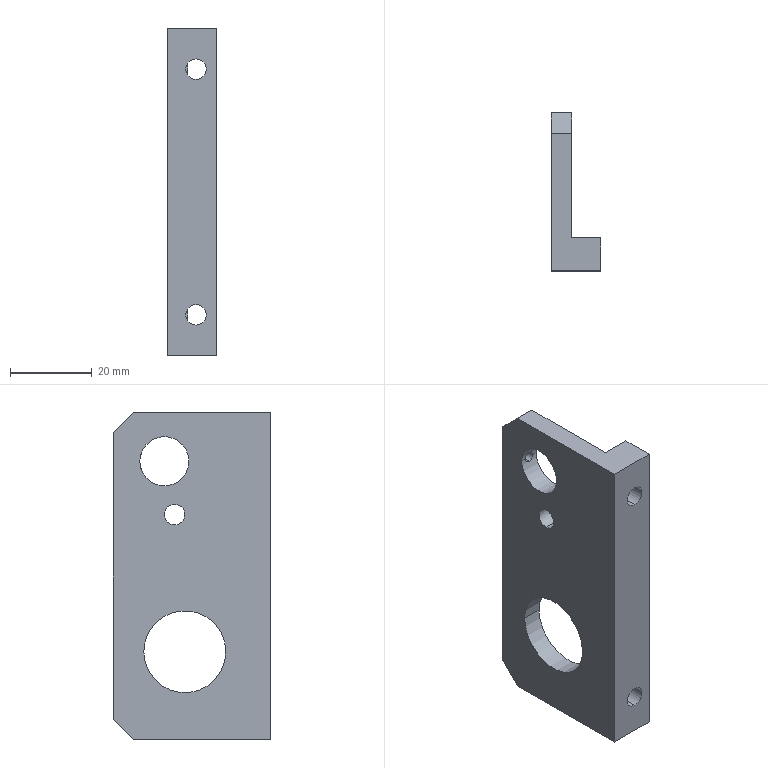Component | SolidWorks | A0116-1 | 1 solid | 24 faces | box 12 x 38.5 x 80 mm | volume 17156 mm3 | cylinder 12 | plane 10 | cone 2 | commonest cylinder face diameters 5 x6 2.5 x2 12 x2 20 x2
build123d program:
from build123d import *

# Parameters (mm, degrees)
BOSS_EXTRUDE1_DEPTH    = 40
SKETCH2_R              = 10
SKETCH2_R_2            = 6
CUT_EXTRUDE1_DEPTH     = 56.958
CHAMFER1_SIZE          = 5
M6_TAPPED_HOLE1_D      = 5
M6_TAPPED_HOLE1_DEPTH  = 17
M6_TAPPED_HOLE1_TIP    = 1.502
M3_TAPPED_HOLE1_REACH  = 58.8
M3_TAPPED_HOLE1_BORE_R = 1.25
M5_TAPPED_HOLE1_D      = 5
M5_TAPPED_HOLE1_DEPTH  = 14
M5_TAPPED_HOLE1_TIP    = 1.502


with BuildPart() as part:
    # Sketch1 → Boss-Extrude1 (new, symmetric)
    with BuildSketch(Plane.XY):
        Polygon((-12, 0), (0, 0), (0, -38.5), (-5, -38.5), (-5, -8), (-12, -8), align=None)
    extrude(amount=BOSS_EXTRUDE1_DEPTH, both=True)

    # Sketch2 → Cut-Extrude1 (cut, through all)
    with BuildSketch(Plane.ZY.offset(5)):
        with Locations(Location((-18.5, -21, 0), (0, 0, 270))):
            Circle(SKETCH2_R)
        with Locations(Location((28, -26, 0), (0, 0, 270))):
            Circle(SKETCH2_R_2)
    extrude(amount=-CUT_EXTRUDE1_DEPTH, mode=Mode.SUBTRACT)

    # Chamfer1
    chamfer1_edges = [part.edges().sort_by_distance(p)[0] for p in [
        (-2.5, -38.5, 40),
        (-2.5, -38.5, -40),
    ]]
    chamfer(chamfer1_edges, length=CHAMFER1_SIZE)

    # M6 Tapped Hole1
    with Locations(Plane(origin=(0, 0, 0), x_dir=(1, 0, 0), z_dir=(0, 1, 0))):
        with Locations((-7, 30), (-7, -30)):
            Hole(M6_TAPPED_HOLE1_D / 2, depth=M6_TAPPED_HOLE1_DEPTH)
            with Locations((0, 0, -(M6_TAPPED_HOLE1_DEPTH + M6_TAPPED_HOLE1_TIP / 2))):  # 118° drill point
                Cone(0, M6_TAPPED_HOLE1_D / 2, M6_TAPPED_HOLE1_TIP, mode=Mode.SUBTRACT)

    # M3 Tapped Hole1 bore → M3 Tapped Hole1 (cut, up to next)
    with BuildSketch(Plane(origin=(0, -38.5, 0), x_dir=(-1, 0, 0), z_dir=(0, -1, 0)), mode=Mode.PRIVATE) as m3_tapped_hole1_sk1:
        with Locations((2.5, -28)):
            Circle(M3_TAPPED_HOLE1_BORE_R)
    m3_tapped_hole1_tool1 = extrude(m3_tapped_hole1_sk1.sketch, amount=-M3_TAPPED_HOLE1_REACH, mode=Mode.PRIVATE) & part.part
    add(m3_tapped_hole1_tool1.solids().sort_by_distance((-2.5, -38.5, 28))[0], mode=Mode.SUBTRACT)

    # M5 Tapped Hole1
    with Locations(Plane(origin=(0, 0, 0), x_dir=(0, 0, -1), z_dir=(1, 0, 0))):
        with Locations((-15, -23.5)):
            Hole(M5_TAPPED_HOLE1_D / 2, depth=M5_TAPPED_HOLE1_DEPTH)
            with Locations((0, 0, -(M5_TAPPED_HOLE1_DEPTH + M5_TAPPED_HOLE1_TIP / 2))):  # 118° drill point
                Cone(0, M5_TAPPED_HOLE1_D / 2, M5_TAPPED_HOLE1_TIP, mode=Mode.SUBTRACT)


solid = part.part

# Placed as in the assembly
solid = solid.moved(Location((-32.619, 0, 60), (0, 0, 180)))
STEP:
#1=COLOUR_RGB('',0.7922,0.8196,0.9333);
#2=FILL_AREA_STYLE_COLOUR('',#1);
#3=FILL_AREA_STYLE('',(#2));
#4=SURFACE_STYLE_FILL_AREA(#3);
#5=SURFACE_SIDE_STYLE('',(#4));
#6=SURFACE_STYLE_USAGE(.BOTH.,#5);
#7=PRESENTATION_STYLE_ASSIGNMENT((#6));
#8=CARTESIAN_POINT('',(-1.087,0.9252,3.051));
#9=VERTEX_POINT('',#8);
#10=CARTESIAN_POINT('',(-1.087,0.9252,2.854));
#11=VERTEX_POINT('',#10);
#12=CARTESIAN_POINT('',(-1.087,0.9252,2.953));
#13=DIRECTION('',(-1.,-0.,0.));
#14=DIRECTION('',(0.,-1.,0.));
#15=AXIS2_PLACEMENT_3D('',#12,#13,#14);
#16=CIRCLE('',#15,0.09843);
#17=EDGE_CURVE('',#9,#11,#16,.T.);
#18=ORIENTED_EDGE('',*,*,#17,.F.);
#19=CARTESIAN_POINT('',(-1.284,0.9252,3.051));
#20=VERTEX_POINT('',#19);
#21=CARTESIAN_POINT('',(-1.284,0.9252,3.051));
#22=DIRECTION('',(-1.,-0.,0.));
#23=VECTOR('',#22,39.37);
#24=LINE('',#21,#23);
#25=EDGE_CURVE('',#9,#20,#24,.T.);
#26=ORIENTED_EDGE('',*,*,#25,.T.);
#27=CARTESIAN_POINT('',(-1.284,0.9252,2.854));
#28=VERTEX_POINT('',#27);
#29=CARTESIAN_POINT('',(-1.284,0.9252,2.953));
#30=DIRECTION('',(-1.,-0.,0.));
#31=DIRECTION('',(-0.,0.,-1.));
#32=AXIS2_PLACEMENT_3D('',#29,#30,#31);
#33=CIRCLE('',#32,0.09843);
#34=EDGE_CURVE('',#20,#28,#33,.T.);
#35=ORIENTED_EDGE('',*,*,#34,.T.);
#36=CARTESIAN_POINT('',(-1.284,0.9252,2.854));
#37=DIRECTION('',(-1.,-0.,0.));
#38=VECTOR('',#37,39.37);
#39=LINE('',#36,#38);
#40=EDGE_CURVE('',#11,#28,#39,.T.);
#41=ORIENTED_EDGE('',*,*,#40,.F.);
#42=EDGE_LOOP('',(#18,#26,#35,#41));
#43=FACE_OUTER_BOUND('',#42,.T.);
#44=CARTESIAN_POINT('',(-1.284,0.9252,2.953));
#45=DIRECTION('',(-1.,-0.,0.));
#46=DIRECTION('',(-0.,0.,-1.));
#47=AXIS2_PLACEMENT_3D('',#44,#45,#46);
#48=CYLINDRICAL_SURFACE('',#47,0.09843);
#49=ADVANCED_FACE('',(#43),#48,.F.);
#50=CARTESIAN_POINT('',(-1.186,1.255,3.514));
#51=VERTEX_POINT('',#50);
#52=CARTESIAN_POINT('',(-1.137,1.26,3.465));
#53=VERTEX_POINT('',#52);
#54=CARTESIAN_POINT('',(-1.186,1.255,3.514));
#55=CARTESIAN_POINT('',(-1.183,1.255,3.514));
#56=CARTESIAN_POINT('',(-1.179,1.255,3.513));
#57=CARTESIAN_POINT('',(-1.173,1.255,3.512));
#58=CARTESIAN_POINT('',(-1.17,1.255,3.511));
#59=CARTESIAN_POINT('',(-1.161,1.256,3.508));
#60=CARTESIAN_POINT('',(-1.156,1.257,3.504));
#61=CARTESIAN_POINT('',(-1.146,1.258,3.495));
#62=CARTESIAN_POINT('',(-1.143,1.259,3.489));
#63=CARTESIAN_POINT('',(-1.138,1.26,3.477));
#64=CARTESIAN_POINT('',(-1.137,1.26,3.471));
#65=CARTESIAN_POINT('',(-1.137,1.26,3.465));
#66=B_SPLINE_CURVE_WITH_KNOTS('',3,(#54,#55,#56,#57,#58,#59,#60,#61,#62,#63,#64,#65),.UNSPECIFIED.,.F.,.F.,(4,2,2,2,2,4),(0.00196,0.002205,0.00245,0.002939,0.003429,0.003919),.UNSPECIFIED.);
#67=EDGE_CURVE('',#51,#53,#66,.T.);
#68=ORIENTED_EDGE('',*,*,#67,.F.);
#69=CARTESIAN_POINT('',(-1.186,1.516,3.514));
#70=VERTEX_POINT('',#69);
#71=CARTESIAN_POINT('',(-1.186,1.516,3.514));
#72=DIRECTION('',(-0.,1.,-0.));
#73=VECTOR('',#72,39.37);
#74=LINE('',#71,#73);
#75=EDGE_CURVE('',#51,#70,#74,.T.);
#76=ORIENTED_EDGE('',*,*,#75,.T.);
#77=CARTESIAN_POINT('',(-1.186,1.516,3.415));
#78=VERTEX_POINT('',#77);
#79=CARTESIAN_POINT('',(-1.186,1.516,3.465));
#80=DIRECTION('',(-0.,1.,-0.));
#81=DIRECTION('',(-0.,0.,-1.));
#82=AXIS2_PLACEMENT_3D('',#79,#80,#81);
#83=CIRCLE('',#82,0.04921);
#84=EDGE_CURVE('',#70,#78,#83,.T.);
#85=ORIENTED_EDGE('',*,*,#84,.T.);
#86=CARTESIAN_POINT('',(-1.186,1.255,3.415));
#87=VERTEX_POINT('',#86);
#88=CARTESIAN_POINT('',(-1.186,1.516,3.415));
#89=DIRECTION('',(-0.,1.,-0.));
#90=VECTOR('',#89,39.37);
#91=LINE('',#88,#90);
#92=EDGE_CURVE('',#87,#78,#91,.T.);
#93=ORIENTED_EDGE('',*,*,#92,.F.);
#94=CARTESIAN_POINT('',(-1.137,1.26,3.465));
#95=CARTESIAN_POINT('',(-1.137,1.26,3.458));
#96=CARTESIAN_POINT('',(-1.138,1.26,3.452));
#97=CARTESIAN_POINT('',(-1.143,1.259,3.44));
#98=CARTESIAN_POINT('',(-1.146,1.258,3.434));
#99=CARTESIAN_POINT('',(-1.156,1.257,3.425));
#100=CARTESIAN_POINT('',(-1.161,1.256,3.422));
#101=CARTESIAN_POINT('',(-1.173,1.255,3.417));
#102=CARTESIAN_POINT('',(-1.179,1.255,3.415));
#103=CARTESIAN_POINT('',(-1.186,1.255,3.415));
#104=B_SPLINE_CURVE_WITH_KNOTS('',3,(#94,#95,#96,#97,#98,#99,#100,#101,#102,#103),.UNSPECIFIED.,.F.,.F.,(4,2,2,2,4),(0.003919,0.004409,0.004899,0.005388,0.005878),.UNSPECIFIED.);
#105=EDGE_CURVE('',#53,#87,#104,.T.);
#106=ORIENTED_EDGE('',*,*,#105,.F.);
#107=EDGE_LOOP('',(#68,#76,#85,#93,#106));
#108=FACE_OUTER_BOUND('',#107,.T.);
#109=CARTESIAN_POINT('',(-1.186,1.516,3.465));
#110=DIRECTION('',(-0.,1.,-0.));
#111=DIRECTION('',(-0.,0.,-1.));
#112=AXIS2_PLACEMENT_3D('',#109,#110,#111);
#113=CYLINDRICAL_SURFACE('',#112,0.04921);
#114=ADVANCED_FACE('',(#108),#113,.F.);
#115=CARTESIAN_POINT('',(-1.009,0.315,1.083));
#116=VERTEX_POINT('',#115);
#117=CARTESIAN_POINT('',(-1.009,0.315,1.28));
#118=VERTEX_POINT('',#117);
#119=CARTESIAN_POINT('',(-1.009,0.315,1.181));
#120=DIRECTION('',(0.,-1.,0.));
#121=DIRECTION('',(1.,0.,-0.));
#122=AXIS2_PLACEMENT_3D('',#119,#120,#121);
#123=CIRCLE('',#122,0.09843);
#124=EDGE_CURVE('',#116,#118,#123,.T.);
#125=ORIENTED_EDGE('',*,*,#124,.F.);
#126=CARTESIAN_POINT('',(-1.009,-0.,1.083));
#127=VERTEX_POINT('',#126);
#128=CARTESIAN_POINT('',(-1.009,-0.,1.083));
#129=DIRECTION('',(0.,-1.,0.));
#130=VECTOR('',#129,39.37);
#131=LINE('',#128,#130);
#132=EDGE_CURVE('',#116,#127,#131,.T.);
#133=ORIENTED_EDGE('',*,*,#132,.T.);
#134=CARTESIAN_POINT('',(-1.009,-0.,1.28));
#135=VERTEX_POINT('',#134);
#136=CARTESIAN_POINT('',(-1.009,-0.,1.181));
#137=DIRECTION('',(0.,-1.,0.));
#138=DIRECTION('',(0.,0.,1.));
#139=AXIS2_PLACEMENT_3D('',#136,#137,#138);
#140=CIRCLE('',#139,0.09843);
#141=EDGE_CURVE('',#127,#135,#140,.T.);
#142=ORIENTED_EDGE('',*,*,#141,.T.);
#143=CARTESIAN_POINT('',(-1.009,-0.,1.28));
#144=DIRECTION('',(0.,-1.,0.));
#145=VECTOR('',#144,39.37);
#146=LINE('',#143,#145);
#147=EDGE_CURVE('',#118,#135,#146,.T.);
#148=ORIENTED_EDGE('',*,*,#147,.F.);
#149=EDGE_LOOP('',(#125,#133,#142,#148));
#150=FACE_OUTER_BOUND('',#149,.T.);
#151=CARTESIAN_POINT('',(-1.009,-0.,1.181));
#152=DIRECTION('',(0.,-1.,0.));
#153=DIRECTION('',(0.,0.,1.));
#154=AXIS2_PLACEMENT_3D('',#151,#152,#153);
#155=CYLINDRICAL_SURFACE('',#154,0.09843);
#156=ADVANCED_FACE('',(#150),#155,.F.);
#157=CARTESIAN_POINT('',(-1.009,0.315,3.445));
#158=VERTEX_POINT('',#157);
#159=CARTESIAN_POINT('',(-1.009,0.315,3.642));
#160=VERTEX_POINT('',#159);
#161=CARTESIAN_POINT('',(-1.009,0.315,3.543));
#162=DIRECTION('',(0.,-1.,0.));
#163=DIRECTION('',(1.,0.,-0.));
#164=AXIS2_PLACEMENT_3D('',#161,#162,#163);
#165=CIRCLE('',#164,0.09843);
#166=EDGE_CURVE('',#158,#160,#165,.T.);
#167=ORIENTED_EDGE('',*,*,#166,.F.);
#168=CARTESIAN_POINT('',(-1.009,-0.,3.445));
#169=VERTEX_POINT('',#168);
#170=CARTESIAN_POINT('',(-1.009,-0.,3.445));
#171=DIRECTION('',(0.,-1.,0.));
#172=VECTOR('',#171,39.37);
#173=LINE('',#170,#172);
#174=EDGE_CURVE('',#158,#169,#173,.T.);
#175=ORIENTED_EDGE('',*,*,#174,.T.);
#176=CARTESIAN_POINT('',(-1.009,-0.,3.642));
#177=VERTEX_POINT('',#176);
#178=CARTESIAN_POINT('',(-1.009,-0.,3.543));
#179=DIRECTION('',(0.,-1.,0.));
#180=DIRECTION('',(0.,0.,1.));
#181=AXIS2_PLACEMENT_3D('',#178,#179,#180);
#182=CIRCLE('',#181,0.09843);
#183=EDGE_CURVE('',#169,#177,#182,.T.);
#184=ORIENTED_EDGE('',*,*,#183,.T.);
#185=CARTESIAN_POINT('',(-1.009,-0.,3.642));
#186=DIRECTION('',(0.,-1.,0.));
#187=VECTOR('',#186,39.37);
#188=LINE('',#185,#187);
#189=EDGE_CURVE('',#160,#177,#188,.T.);
#190=ORIENTED_EDGE('',*,*,#189,.F.);
#191=EDGE_LOOP('',(#167,#175,#184,#190));
#192=FACE_OUTER_BOUND('',#191,.T.);
#193=CARTESIAN_POINT('',(-1.009,-0.,3.543));
#194=DIRECTION('',(0.,-1.,0.));
#195=DIRECTION('',(0.,0.,1.));
#196=AXIS2_PLACEMENT_3D('',#193,#194,#195);
#197=CYLINDRICAL_SURFACE('',#196,0.09843);
#198=ADVANCED_FACE('',(#192),#197,.F.);
#199=CARTESIAN_POINT('',(-1.284,0.7874,3.465));
#200=VERTEX_POINT('',#199);
#201=CARTESIAN_POINT('',(-1.284,1.26,3.465));
#202=VERTEX_POINT('',#201);
#203=CARTESIAN_POINT('',(-1.284,1.024,3.465));
#204=DIRECTION('',(1.,0.,-0.));
#205=DIRECTION('',(-0.,1.,0.));
#206=AXIS2_PLACEMENT_3D('',#203,#204,#205);
#207=CIRCLE('',#206,0.2362);
#208=EDGE_CURVE('',#200,#202,#207,.T.);
#209=ORIENTED_EDGE('',*,*,#208,.F.);
#210=CARTESIAN_POINT('',(-1.087,0.7874,3.465));
#211=VERTEX_POINT('',#210);
#212=CARTESIAN_POINT('',(-1.284,0.7874,3.465));
#213=DIRECTION('',(1.,0.,-0.));
#214=VECTOR('',#213,39.37);
#215=LINE('',#212,#214);
#216=EDGE_CURVE('',#200,#211,#215,.T.);
#217=ORIENTED_EDGE('',*,*,#216,.T.);
#218=CARTESIAN_POINT('',(-1.087,1.26,3.465));
#219=VERTEX_POINT('',#218);
#220=CARTESIAN_POINT('',(-1.087,1.024,3.465));
#221=DIRECTION('',(1.,0.,-0.));
#222=DIRECTION('',(-0.,1.,0.));
#223=AXIS2_PLACEMENT_3D('',#220,#221,#222);
#224=CIRCLE('',#223,0.2362);
#225=EDGE_CURVE('',#211,#219,#224,.T.);
#226=ORIENTED_EDGE('',*,*,#225,.T.);
#227=CARTESIAN_POINT('',(-1.284,1.26,3.465));
#228=DIRECTION('',(1.,0.,-0.));
#229=VECTOR('',#228,39.37);
#230=LINE('',#227,#229);
#231=EDGE_CURVE('',#53,#219,#230,.T.);
#232=ORIENTED_EDGE('',*,*,#231,.F.);
#233=ORIENTED_EDGE('',*,*,#105,.T.);
#234=CARTESIAN_POINT('',(-1.235,1.26,3.465));
#235=VERTEX_POINT('',#234);
#236=CARTESIAN_POINT('',(-1.186,1.255,3.415));
#237=CARTESIAN_POINT('',(-1.192,1.255,3.415));
#238=CARTESIAN_POINT('',(-1.199,1.255,3.417));
#239=CARTESIAN_POINT('',(-1.211,1.256,3.422));
#240=CARTESIAN_POINT('',(-1.216,1.257,3.425));
#241=CARTESIAN_POINT('',(-1.225,1.258,3.434));
#242=CARTESIAN_POINT('',(-1.229,1.259,3.44));
#243=CARTESIAN_POINT('',(-1.234,1.26,3.452));
#244=CARTESIAN_POINT('',(-1.235,1.26,3.458));
#245=CARTESIAN_POINT('',(-1.235,1.26,3.465));
#246=B_SPLINE_CURVE_WITH_KNOTS('',3,(#236,#237,#238,#239,#240,#241,#242,#243,#244,#245),.UNSPECIFIED.,.F.,.F.,(4,2,2,2,4),(0.005878,0.006368,0.006857,0.007347,0.007837),.UNSPECIFIED.);
#247=EDGE_CURVE('',#87,#235,#246,.T.);
#248=ORIENTED_EDGE('',*,*,#247,.T.);
#249=CARTESIAN_POINT('',(-1.284,1.26,3.465));
#250=DIRECTION('',(1.,0.,-0.));
#251=VECTOR('',#250,39.37);
#252=LINE('',#249,#251);
#253=EDGE_CURVE('',#202,#235,#252,.T.);
#254=ORIENTED_EDGE('',*,*,#253,.F.);
#255=EDGE_LOOP('',(#209,#217,#226,#232,#233,#248,#254));
#256=FACE_OUTER_BOUND('',#255,.T.);
#257=CARTESIAN_POINT('',(-1.284,1.024,3.465));
#258=DIRECTION('',(1.,0.,-0.));
#259=DIRECTION('',(-0.,1.,0.));
#260=AXIS2_PLACEMENT_3D('',#257,#258,#259);
#261=CYLINDRICAL_SURFACE('',#260,0.2362);
#262=ADVANCED_FACE('',(#256),#261,.F.);
#263=CARTESIAN_POINT('',(-1.284,0.4331,1.634));
#264=VERTEX_POINT('',#263);
#265=CARTESIAN_POINT('',(-1.284,1.22,1.634));
#266=VERTEX_POINT('',#265);
#267=CARTESIAN_POINT('',(-1.284,0.8268,1.634));
#268=DIRECTION('',(1.,0.,-0.));
#269=DIRECTION('',(-0.,1.,0.));
#270=AXIS2_PLACEMENT_3D('',#267,#268,#269);
#271=CIRCLE('',#270,0.3937);
#272=EDGE_CURVE('',#264,#266,#271,.T.);
#273=ORIENTED_EDGE('',*,*,#272,.F.);
#274=CARTESIAN_POINT('',(-1.087,0.4331,1.634));
#275=VERTEX_POINT('',#274);
#276=CARTESIAN_POINT('',(-1.284,0.4331,1.634));
#277=DIRECTION('',(1.,0.,-0.));
#278=VECTOR('',#277,39.37);
#279=LINE('',#276,#278);
#280=EDGE_CURVE('',#264,#275,#279,.T.);
#281=ORIENTED_EDGE('',*,*,#280,.T.);
#282=CARTESIAN_POINT('',(-1.087,1.22,1.634));
#283=VERTEX_POINT('',#282);
#284=CARTESIAN_POINT('',(-1.087,0.8268,1.634));
#285=DIRECTION('',(1.,0.,-0.));
#286=DIRECTION('',(-0.,1.,0.));
#287=AXIS2_PLACEMENT_3D('',#284,#285,#286);
#288=CIRCLE('',#287,0.3937);
#289=EDGE_CURVE('',#275,#283,#288,.T.);
#290=ORIENTED_EDGE('',*,*,#289,.T.);
#291=CARTESIAN_POINT('',(-1.284,1.22,1.634));
#292=DIRECTION('',(1.,0.,-0.));
#293=VECTOR('',#292,39.37);
#294=LINE('',#291,#293);
#295=EDGE_CURVE('',#266,#283,#294,.T.);
#296=ORIENTED_EDGE('',*,*,#295,.F.);
#297=EDGE_LOOP('',(#273,#281,#290,#296));
#298=FACE_OUTER_BOUND('',#297,.T.);
#299=CARTESIAN_POINT('',(-1.284,0.8268,1.634));
#300=DIRECTION('',(1.,0.,-0.));
#301=DIRECTION('',(-0.,1.,0.));
#302=AXIS2_PLACEMENT_3D('',#299,#300,#301);
#303=CYLINDRICAL_SURFACE('',#302,0.3937);
#304=ADVANCED_FACE('',(#298),#303,.F.);
#305=CARTESIAN_POINT('',(-0.8118,-0.,0.7874));
#306=VERTEX_POINT('',#305);
#307=CARTESIAN_POINT('',(-0.8118,0.315,0.7874));
#308=VERTEX_POINT('',#307);
#309=CARTESIAN_POINT('',(-0.8118,0.315,0.7874));
#310=DIRECTION('',(-0.,1.,-0.));
#311=VECTOR('',#310,39.37);
#312=LINE('',#309,#311);
#313=EDGE_CURVE('',#306,#308,#312,.T.);
#314=ORIENTED_EDGE('',*,*,#313,.T.);
#315=CARTESIAN_POINT('',(-0.8118,0.315,3.937));
#316=VERTEX_POINT('',#315);
#317=CARTESIAN_POINT('',(-0.8118,0.315,3.937));
#318=DIRECTION('',(-0.,-0.,-1.));
#319=VECTOR('',#318,39.37);
#320=LINE('',#317,#319);
#321=EDGE_CURVE('',#316,#308,#320,.T.);
#322=ORIENTED_EDGE('',*,*,#321,.F.);
#323=CARTESIAN_POINT('',(-0.8118,-0.,3.937));
#324=VERTEX_POINT('',#323);
#325=CARTESIAN_POINT('',(-0.8118,0.315,3.937));
#326=DIRECTION('',(-0.,1.,-0.));
#327=VECTOR('',#326,39.37);
#328=LINE('',#325,#327);
#329=EDGE_CURVE('',#324,#316,#328,.T.);
#330=ORIENTED_EDGE('',*,*,#329,.F.);
#331=CARTESIAN_POINT('',(-0.8118,-0.,3.937));
#332=DIRECTION('',(-0.,-0.,-1.));
#333=VECTOR('',#332,39.37);
#334=LINE('',#331,#333);
#335=EDGE_CURVE('',#324,#306,#334,.T.);
#336=ORIENTED_EDGE('',*,*,#335,.T.);
#337=EDGE_LOOP('',(#314,#322,#330,#336));
#338=FACE_OUTER_BOUND('',#337,.T.);
#339=CARTESIAN_POINT('',(-0.8118,0.315,3.937));
#340=DIRECTION('',(-1.,-0.,0.));
#341=DIRECTION('',(-0.,-0.,-1.));
#342=AXIS2_PLACEMENT_3D('',#339,#340,#341);
#343=PLANE('',#342);
#344=ADVANCED_FACE('',(#338),#343,.F.);
#345=CARTESIAN_POINT('',(-1.087,0.315,1.122));
#346=VERTEX_POINT('',#345);
#347=CARTESIAN_POINT('',(-1.087,0.315,0.7874));
#348=VERTEX_POINT('',#347);
#349=CARTESIAN_POINT('',(-1.087,0.315,3.937));
#350=DIRECTION('',(-0.,-0.,-1.));
#351=VECTOR('',#350,39.37);
#352=LINE('',#349,#351);
#353=EDGE_CURVE('',#346,#348,#352,.T.);
#354=ORIENTED_EDGE('',*,*,#353,.F.);
#355=CARTESIAN_POINT('',(-1.009,0.315,1.181));
#356=DIRECTION('',(0.,-1.,0.));
#357=DIRECTION('',(1.,0.,-0.));
#358=AXIS2_PLACEMENT_3D('',#355,#356,#357);
#359=CIRCLE('',#358,0.09843);
#360=EDGE_CURVE('',#346,#116,#359,.T.);
#361=ORIENTED_EDGE('',*,*,#360,.T.);
#362=ORIENTED_EDGE('',*,*,#124,.T.);
#363=CARTESIAN_POINT('',(-1.087,0.315,1.24));
#364=VERTEX_POINT('',#363);
#365=CARTESIAN_POINT('',(-1.009,0.315,1.181));
#366=DIRECTION('',(0.,-1.,0.));
#367=DIRECTION('',(1.,0.,-0.));
#368=AXIS2_PLACEMENT_3D('',#365,#366,#367);
#369=CIRCLE('',#368,0.09843);
#370=EDGE_CURVE('',#118,#364,#369,.T.);
#371=ORIENTED_EDGE('',*,*,#370,.T.);
#372=CARTESIAN_POINT('',(-1.087,0.315,3.484));
#373=VERTEX_POINT('',#372);
#374=CARTESIAN_POINT('',(-1.087,0.315,3.937));
#375=DIRECTION('',(-0.,-0.,-1.));
#376=VECTOR('',#375,39.37);
#377=LINE('',#374,#376);
#378=EDGE_CURVE('',#373,#364,#377,.T.);
#379=ORIENTED_EDGE('',*,*,#378,.F.);
#380=CARTESIAN_POINT('',(-1.009,0.315,3.543));
#381=DIRECTION('',(0.,-1.,0.));
#382=DIRECTION('',(1.,0.,-0.));
#383=AXIS2_PLACEMENT_3D('',#380,#381,#382);
#384=CIRCLE('',#383,0.09843);
#385=EDGE_CURVE('',#373,#158,#384,.T.);
#386=ORIENTED_EDGE('',*,*,#385,.T.);
#387=ORIENTED_EDGE('',*,*,#166,.T.);
#388=CARTESIAN_POINT('',(-1.087,0.315,3.602));
#389=VERTEX_POINT('',#388);
#390=CARTESIAN_POINT('',(-1.009,0.315,3.543));
#391=DIRECTION('',(0.,-1.,0.));
#392=DIRECTION('',(1.,0.,-0.));
#393=AXIS2_PLACEMENT_3D('',#390,#391,#392);
#394=CIRCLE('',#393,0.09843);
#395=EDGE_CURVE('',#160,#389,#394,.T.);
#396=ORIENTED_EDGE('',*,*,#395,.T.);
#397=CARTESIAN_POINT('',(-1.087,0.315,3.937));
#398=VERTEX_POINT('',#397);
#399=CARTESIAN_POINT('',(-1.087,0.315,3.937));
#400=DIRECTION('',(-0.,-0.,-1.));
#401=VECTOR('',#400,39.37);
#402=LINE('',#399,#401);
#403=EDGE_CURVE('',#398,#389,#402,.T.);
#404=ORIENTED_EDGE('',*,*,#403,.F.);
#405=CARTESIAN_POINT('',(-1.087,0.315,3.937));
#406=DIRECTION('',(-1.,-0.,0.));
#407=VECTOR('',#406,39.37);
#408=LINE('',#405,#407);
#409=EDGE_CURVE('',#316,#398,#408,.T.);
#410=ORIENTED_EDGE('',*,*,#409,.F.);
#411=ORIENTED_EDGE('',*,*,#321,.T.);
#412=CARTESIAN_POINT('',(-1.087,0.315,0.7874));
#413=DIRECTION('',(-1.,-0.,0.));
#414=VECTOR('',#413,39.37);
#415=LINE('',#412,#414);
#416=EDGE_CURVE('',#308,#348,#415,.T.);
#417=ORIENTED_EDGE('',*,*,#416,.T.);
#418=EDGE_LOOP('',(#354,#361,#362,#371,#379,#386,#387,#396,#404,#410,#411,#417));
#419=FACE_OUTER_BOUND('',#418,.T.);
#420=CARTESIAN_POINT('',(-1.087,0.315,3.937));
#421=DIRECTION('',(0.,-1.,0.));
#422=DIRECTION('',(1.,0.,-0.));
#423=AXIS2_PLACEMENT_3D('',#420,#421,#422);
#424=PLANE('',#423);
#425=ADVANCED_FACE('',(#419),#424,.F.);
#426=CARTESIAN_POINT('',(-1.087,0.9252,2.953));
#427=DIRECTION('',(-1.,-0.,0.));
#428=DIRECTION('',(0.,-1.,0.));
#429=AXIS2_PLACEMENT_3D('',#426,#427,#428);
#430=CIRCLE('',#429,0.09843);
#431=EDGE_CURVE('',#11,#9,#430,.T.);
#432=ORIENTED_EDGE('',*,*,#431,.T.);
#433=ORIENTED_EDGE('',*,*,#17,.T.);
#434=EDGE_LOOP('',(#432,#433));
#435=FACE_BOUND('',#434,.T.);
#436=CARTESIAN_POINT('',(-1.087,1.024,3.465));
#437=DIRECTION('',(1.,0.,-0.));
#438=DIRECTION('',(-0.,1.,0.));
#439=AXIS2_PLACEMENT_3D('',#436,#437,#438);
#440=CIRCLE('',#439,0.2362);
#441=EDGE_CURVE('',#219,#211,#440,.T.);
#442=ORIENTED_EDGE('',*,*,#441,.F.);
#443=ORIENTED_EDGE('',*,*,#225,.F.);
#444=EDGE_LOOP('',(#442,#443));
#445=FACE_BOUND('',#444,.T.);
#446=CARTESIAN_POINT('',(-1.087,0.8268,1.634));
#447=DIRECTION('',(1.,0.,-0.));
#448=DIRECTION('',(-0.,1.,0.));
#449=AXIS2_PLACEMENT_3D('',#446,#447,#448);
#450=CIRCLE('',#449,0.3937);
#451=EDGE_CURVE('',#283,#275,#450,.T.);
#452=ORIENTED_EDGE('',*,*,#451,.F.);
#453=ORIENTED_EDGE('',*,*,#289,.F.);
#454=EDGE_LOOP('',(#452,#453));
#455=FACE_BOUND('',#454,.T.);
#456=CARTESIAN_POINT('',(-1.087,0.6693,1.24));
#457=VERTEX_POINT('',#456);
#458=CARTESIAN_POINT('',(-1.087,0.6693,1.122));
#459=VERTEX_POINT('',#458);
#460=CARTESIAN_POINT('',(-1.087,0.6693,1.24));
#461=CARTESIAN_POINT('',(-1.087,0.6727,1.231));
#462=CARTESIAN_POINT('',(-1.087,0.6757,1.221));
#463=CARTESIAN_POINT('',(-1.087,0.6799,1.201));
#464=CARTESIAN_POINT('',(-1.087,0.6811,1.191));
#465=CARTESIAN_POINT('',(-1.087,0.6811,1.176));
#466=CARTESIAN_POINT('',(-1.087,0.6808,1.171));
#467=CARTESIAN_POINT('',(-1.087,0.6797,1.161));
#468=CARTESIAN_POINT('',(-1.087,0.6789,1.156));
#469=CARTESIAN_POINT('',(-1.087,0.6757,1.141));
#470=CARTESIAN_POINT('',(-1.087,0.6727,1.132));
#471=CARTESIAN_POINT('',(-1.087,0.6693,1.122));
#472=B_SPLINE_CURVE_WITH_KNOTS('',3,(#460,#461,#462,#463,#464,#465,#466,#467,#468,#469,#470,#471),.UNSPECIFIED.,.F.,.F.,(4,2,2,2,2,4),(0.00544,0.006204,0.006968,0.00735,0.007733,0.008497),.UNSPECIFIED.);
#473=EDGE_CURVE('',#457,#459,#472,.T.);
#474=ORIENTED_EDGE('',*,*,#473,.T.);
#475=CARTESIAN_POINT('',(-1.087,-0.,1.122));
#476=DIRECTION('',(0.,-1.,0.));
#477=VECTOR('',#476,39.37);
#478=LINE('',#475,#477);
#479=EDGE_CURVE('',#459,#346,#478,.T.);
#480=ORIENTED_EDGE('',*,*,#479,.T.);
#481=ORIENTED_EDGE('',*,*,#353,.T.);
#482=CARTESIAN_POINT('',(-1.087,1.319,0.7874));
#483=VERTEX_POINT('',#482);
#484=CARTESIAN_POINT('',(-1.087,1.516,0.7874));
#485=DIRECTION('',(-0.,1.,-0.));
#486=VECTOR('',#485,39.37);
#487=LINE('',#484,#486);
#488=EDGE_CURVE('',#348,#483,#487,.T.);
#489=ORIENTED_EDGE('',*,*,#488,.T.);
#490=CARTESIAN_POINT('',(-1.087,1.516,0.9843));
#491=VERTEX_POINT('',#490);
#492=CARTESIAN_POINT('',(-1.087,1.516,0.9843));
#493=DIRECTION('',(0.,0.7071,0.7071));
#494=VECTOR('',#493,39.37);
#495=LINE('',#492,#494);
#496=EDGE_CURVE('',#483,#491,#495,.T.);
#497=ORIENTED_EDGE('',*,*,#496,.T.);
#498=CARTESIAN_POINT('',(-1.087,1.516,3.74));
#499=VERTEX_POINT('',#498);
#500=CARTESIAN_POINT('',(-1.087,1.516,3.937));
#501=DIRECTION('',(-0.,-0.,-1.));
#502=VECTOR('',#501,39.37);
#503=LINE('',#500,#502);
#504=EDGE_CURVE('',#499,#491,#503,.T.);
#505=ORIENTED_EDGE('',*,*,#504,.F.);
#506=CARTESIAN_POINT('',(-1.087,1.319,3.937));
#507=VERTEX_POINT('',#506);
#508=CARTESIAN_POINT('',(-1.087,1.319,3.937));
#509=DIRECTION('',(0.,-0.7071,0.7071));
#510=VECTOR('',#509,39.37);
#511=LINE('',#508,#510);
#512=EDGE_CURVE('',#499,#507,#511,.T.);
#513=ORIENTED_EDGE('',*,*,#512,.T.);
#514=CARTESIAN_POINT('',(-1.087,1.516,3.937));
#515=DIRECTION('',(-0.,1.,-0.));
#516=VECTOR('',#515,39.37);
#517=LINE('',#514,#516);
#518=EDGE_CURVE('',#398,#507,#517,.T.);
#519=ORIENTED_EDGE('',*,*,#518,.F.);
#520=ORIENTED_EDGE('',*,*,#403,.T.);
#521=CARTESIAN_POINT('',(-1.087,0.6693,3.602));
#522=VERTEX_POINT('',#521);
#523=CARTESIAN_POINT('',(-1.087,-0.,3.602));
#524=DIRECTION('',(-0.,1.,-0.));
#525=VECTOR('',#524,39.37);
#526=LINE('',#523,#525);
#527=EDGE_CURVE('',#389,#522,#526,.T.);
#528=ORIENTED_EDGE('',*,*,#527,.T.);
#529=CARTESIAN_POINT('',(-1.087,0.6693,3.484));
#530=VERTEX_POINT('',#529);
#531=CARTESIAN_POINT('',(-1.087,0.6693,3.602));
#532=CARTESIAN_POINT('',(-1.087,0.6727,3.593));
#533=CARTESIAN_POINT('',(-1.087,0.6757,3.583));
#534=CARTESIAN_POINT('',(-1.087,0.6799,3.564));
#535=CARTESIAN_POINT('',(-1.087,0.6811,3.554));
#536=CARTESIAN_POINT('',(-1.087,0.6811,3.538));
#537=CARTESIAN_POINT('',(-1.087,0.6808,3.533));
#538=CARTESIAN_POINT('',(-1.087,0.6797,3.523));
#539=CARTESIAN_POINT('',(-1.087,0.6789,3.518));
#540=CARTESIAN_POINT('',(-1.087,0.6757,3.503));
#541=CARTESIAN_POINT('',(-1.087,0.6727,3.494));
#542=CARTESIAN_POINT('',(-1.087,0.6693,3.484));
#543=B_SPLINE_CURVE_WITH_KNOTS('',3,(#531,#532,#533,#534,#535,#536,#537,#538,#539,#540,#541,#542),.UNSPECIFIED.,.F.,.F.,(4,2,2,2,2,4),(0.00544,0.006204,0.006968,0.00735,0.007733,0.008497),.UNSPECIFIED.);
#544=EDGE_CURVE('',#522,#530,#543,.T.);
#545=ORIENTED_EDGE('',*,*,#544,.T.);
#546=CARTESIAN_POINT('',(-1.087,-0.,3.484));
#547=DIRECTION('',(0.,-1.,0.));
#548=VECTOR('',#547,39.37);
#549=LINE('',#546,#548);
#550=EDGE_CURVE('',#530,#373,#549,.T.);
#551=ORIENTED_EDGE('',*,*,#550,.T.);
#552=ORIENTED_EDGE('',*,*,#378,.T.);
#553=CARTESIAN_POINT('',(-1.087,-0.,1.24));
#554=DIRECTION('',(-0.,1.,-0.));
#555=VECTOR('',#554,39.37);
#556=LINE('',#553,#555);
#557=EDGE_CURVE('',#364,#457,#556,.T.);
#558=ORIENTED_EDGE('',*,*,#557,.T.);
#559=EDGE_LOOP('',(#474,#480,#481,#489,#497,#505,#513,#519,#520,#528,#545,#551,#552,#558));
#560=FACE_OUTER_BOUND('',#559,.T.);
#561=CARTESIAN_POINT('',(-1.087,1.516,3.937));
#562=DIRECTION('',(-1.,-0.,0.));
#563=DIRECTION('',(0.,-1.,0.));
#564=AXIS2_PLACEMENT_3D('',#561,#562,#563);
#565=PLANE('',#564);
#566=ADVANCED_FACE('',(#435,#445,#455,#560),#565,.F.);
#567=CARTESIAN_POINT('',(-1.186,1.516,3.465));
#568=DIRECTION('',(-0.,1.,-0.));
#569=DIRECTION('',(-0.,0.,-1.));
#570=AXIS2_PLACEMENT_3D('',#567,#568,#569);
#571=CIRCLE('',#570,0.04921);
#572=EDGE_CURVE('',#78,#70,#571,.T.);
#573=ORIENTED_EDGE('',*,*,#572,.F.);
#574=ORIENTED_EDGE('',*,*,#84,.F.);
#575=EDGE_LOOP('',(#573,#574));
#576=FACE_BOUND('',#575,.T.);
#577=CARTESIAN_POINT('',(-1.284,1.516,3.74));
#578=VERTEX_POINT('',#577);
#579=CARTESIAN_POINT('',(-1.284,1.516,0.9843));
#580=VERTEX_POINT('',#579);
#581=CARTESIAN_POINT('',(-1.284,1.516,3.937));
#582=DIRECTION('',(-0.,-0.,-1.));
#583=VECTOR('',#582,39.37);
#584=LINE('',#581,#583);
#585=EDGE_CURVE('',#578,#580,#584,.T.);
#586=ORIENTED_EDGE('',*,*,#585,.F.);
#587=CARTESIAN_POINT('',(-1.284,1.516,3.74));
#588=DIRECTION('',(1.,-0.,-0.));
#589=VECTOR('',#588,39.37);
#590=LINE('',#587,#589);
#591=EDGE_CURVE('',#578,#499,#590,.T.);
#592=ORIENTED_EDGE('',*,*,#591,.T.);
#593=ORIENTED_EDGE('',*,*,#504,.T.);
#594=CARTESIAN_POINT('',(-1.284,1.516,0.9843));
#595=DIRECTION('',(-1.,0.,0.));
#596=VECTOR('',#595,39.37);
#597=LINE('',#594,#596);
#598=EDGE_CURVE('',#491,#580,#597,.T.);
#599=ORIENTED_EDGE('',*,*,#598,.T.);
#600=EDGE_LOOP('',(#586,#592,#593,#599));
#601=FACE_OUTER_BOUND('',#600,.T.);
#602=CARTESIAN_POINT('',(-1.284,1.516,3.937));
#603=DIRECTION('',(-0.,-1.,0.));
#604=DIRECTION('',(1.,-0.,-0.));
#605=AXIS2_PLACEMENT_3D('',#602,#603,#604);
#606=PLANE('',#605);
#607=ADVANCED_FACE('',(#576,#601),#606,.F.);
#608=CARTESIAN_POINT('',(-1.284,0.9252,2.953));
#609=DIRECTION('',(-1.,-0.,0.));
#610=DIRECTION('',(-0.,0.,-1.));
#611=AXIS2_PLACEMENT_3D('',#608,#609,#610);
#612=CIRCLE('',#611,0.09843);
#613=EDGE_CURVE('',#28,#20,#612,.T.);
#614=ORIENTED_EDGE('',*,*,#613,.F.);
#615=ORIENTED_EDGE('',*,*,#34,.F.);
#616=EDGE_LOOP('',(#614,#615));
#617=FACE_BOUND('',#616,.T.);
#618=CARTESIAN_POINT('',(-1.284,1.024,3.465));
#619=DIRECTION('',(1.,0.,-0.));
#620=DIRECTION('',(-0.,1.,0.));
#621=AXIS2_PLACEMENT_3D('',#618,#619,#620);
#622=CIRCLE('',#621,0.2362);
#623=EDGE_CURVE('',#202,#200,#622,.T.);
#624=ORIENTED_EDGE('',*,*,#623,.T.);
#625=ORIENTED_EDGE('',*,*,#208,.T.);
#626=EDGE_LOOP('',(#624,#625));
#627=FACE_BOUND('',#626,.T.);
#628=CARTESIAN_POINT('',(-1.284,0.8268,1.634));
#629=DIRECTION('',(1.,0.,-0.));
#630=DIRECTION('',(-0.,1.,0.));
#631=AXIS2_PLACEMENT_3D('',#628,#629,#630);
#632=CIRCLE('',#631,0.3937);
#633=EDGE_CURVE('',#266,#264,#632,.T.);
#634=ORIENTED_EDGE('',*,*,#633,.T.);
#635=ORIENTED_EDGE('',*,*,#272,.T.);
#636=EDGE_LOOP('',(#634,#635));
#637=FACE_BOUND('',#636,.T.);
#638=CARTESIAN_POINT('',(-1.284,1.319,3.937));
#639=VERTEX_POINT('',#638);
#640=CARTESIAN_POINT('',(-1.284,-0.,3.937));
#641=VERTEX_POINT('',#640);
#642=CARTESIAN_POINT('',(-1.284,-0.,3.937));
#643=DIRECTION('',(0.,-1.,0.));
#644=VECTOR('',#643,39.37);
#645=LINE('',#642,#644);
#646=EDGE_CURVE('',#639,#641,#645,.T.);
#647=ORIENTED_EDGE('',*,*,#646,.F.);
#648=CARTESIAN_POINT('',(-1.284,1.319,3.937));
#649=DIRECTION('',(-0.,0.7071,-0.7071));
#650=VECTOR('',#649,39.37);
#651=LINE('',#648,#650);
#652=EDGE_CURVE('',#639,#578,#651,.T.);
#653=ORIENTED_EDGE('',*,*,#652,.T.);
#654=ORIENTED_EDGE('',*,*,#585,.T.);
#655=CARTESIAN_POINT('',(-1.284,1.319,0.7874));
#656=VERTEX_POINT('',#655);
#657=CARTESIAN_POINT('',(-1.284,1.516,0.9843));
#658=DIRECTION('',(-0.,-0.7071,-0.7071));
#659=VECTOR('',#658,39.37);
#660=LINE('',#657,#659);
#661=EDGE_CURVE('',#580,#656,#660,.T.);
#662=ORIENTED_EDGE('',*,*,#661,.T.);
#663=CARTESIAN_POINT('',(-1.284,-0.,0.7874));
#664=VERTEX_POINT('',#663);
#665=CARTESIAN_POINT('',(-1.284,-0.,0.7874));
#666=DIRECTION('',(0.,-1.,0.));
#667=VECTOR('',#666,39.37);
#668=LINE('',#665,#667);
#669=EDGE_CURVE('',#656,#664,#668,.T.);
#670=ORIENTED_EDGE('',*,*,#669,.T.);
#671=CARTESIAN_POINT('',(-1.284,-0.,3.937));
#672=DIRECTION('',(-0.,-0.,-1.));
#673=VECTOR('',#672,39.37);
#674=LINE('',#671,#673);
#675=EDGE_CURVE('',#641,#664,#674,.T.);
#676=ORIENTED_EDGE('',*,*,#675,.F.);
#677=EDGE_LOOP('',(#647,#653,#654,#662,#670,#676));
#678=FACE_OUTER_BOUND('',#677,.T.);
#679=CARTESIAN_POINT('',(-1.284,-0.,3.937));
#680=DIRECTION('',(1.,0.,-0.));
#681=DIRECTION('',(-0.,1.,-0.));
#682=AXIS2_PLACEMENT_3D('',#679,#680,#681);
#683=PLANE('',#682);
#684=ADVANCED_FACE('',(#617,#627,#637,#678),#683,.F.);
#685=CARTESIAN_POINT('',(-1.009,-0.,1.181));
#686=DIRECTION('',(0.,-1.,0.));
#687=DIRECTION('',(0.,0.,1.));
#688=AXIS2_PLACEMENT_3D('',#685,#686,#687);
#689=CIRCLE('',#688,0.09843);
#690=EDGE_CURVE('',#135,#127,#689,.T.);
#691=ORIENTED_EDGE('',*,*,#690,.F.);
#692=ORIENTED_EDGE('',*,*,#141,.F.);
#693=EDGE_LOOP('',(#691,#692));
#694=FACE_BOUND('',#693,.T.);
#695=CARTESIAN_POINT('',(-1.009,-0.,3.543));
#696=DIRECTION('',(0.,-1.,0.));
#697=DIRECTION('',(0.,0.,1.));
#698=AXIS2_PLACEMENT_3D('',#695,#696,#697);
#699=CIRCLE('',#698,0.09843);
#700=EDGE_CURVE('',#177,#169,#699,.T.);
#701=ORIENTED_EDGE('',*,*,#700,.F.);
#702=ORIENTED_EDGE('',*,*,#183,.F.);
#703=EDGE_LOOP('',(#701,#702));
#704=FACE_BOUND('',#703,.T.);
#705=CARTESIAN_POINT('',(-0.8118,-0.,0.7874));
#706=DIRECTION('',(1.,0.,-0.));
#707=VECTOR('',#706,39.37);
#708=LINE('',#705,#707);
#709=EDGE_CURVE('',#664,#306,#708,.T.);
#710=ORIENTED_EDGE('',*,*,#709,.T.);
#711=ORIENTED_EDGE('',*,*,#335,.F.);
#712=CARTESIAN_POINT('',(-0.8118,-0.,3.937));
#713=DIRECTION('',(1.,0.,-0.));
#714=VECTOR('',#713,39.37);
#715=LINE('',#712,#714);
#716=EDGE_CURVE('',#641,#324,#715,.T.);
#717=ORIENTED_EDGE('',*,*,#716,.F.);
#718=ORIENTED_EDGE('',*,*,#675,.T.);
#719=EDGE_LOOP('',(#710,#711,#717,#718));
#720=FACE_OUTER_BOUND('',#719,.T.);
#721=CARTESIAN_POINT('',(-0.8118,-0.,3.937));
#722=DIRECTION('',(-0.,1.,-0.));
#723=DIRECTION('',(-0.,-0.,-1.));
#724=AXIS2_PLACEMENT_3D('',#721,#722,#723);
#725=PLANE('',#724);
#726=ADVANCED_FACE('',(#694,#704,#720),#725,.F.);
#727=ORIENTED_EDGE('',*,*,#518,.T.);
#728=CARTESIAN_POINT('',(-1.284,1.319,3.937));
#729=DIRECTION('',(-1.,0.,0.));
#730=VECTOR('',#729,39.37);
#731=LINE('',#728,#730);
#732=EDGE_CURVE('',#507,#639,#731,.T.);
#733=ORIENTED_EDGE('',*,*,#732,.T.);
#734=ORIENTED_EDGE('',*,*,#646,.T.);
#735=ORIENTED_EDGE('',*,*,#716,.T.);
#736=ORIENTED_EDGE('',*,*,#329,.T.);
#737=ORIENTED_EDGE('',*,*,#409,.T.);
#738=EDGE_LOOP('',(#727,#733,#734,#735,#736,#737));
#739=FACE_OUTER_BOUND('',#738,.T.);
#740=CARTESIAN_POINT('',(-1.284,-0.,3.937));
#741=DIRECTION('',(-0.,-0.,-1.));
#742=DIRECTION('',(1.,0.,-0.));
#743=AXIS2_PLACEMENT_3D('',#740,#741,#742);
#744=PLANE('',#743);
#745=ADVANCED_FACE('',(#739),#744,.F.);
#746=ORIENTED_EDGE('',*,*,#669,.F.);
#747=CARTESIAN_POINT('',(-1.087,1.319,0.7874));
#748=DIRECTION('',(1.,-0.,-0.));
#749=VECTOR('',#748,39.37);
#750=LINE('',#747,#749);
#751=EDGE_CURVE('',#656,#483,#750,.T.);
#752=ORIENTED_EDGE('',*,*,#751,.T.);
#753=ORIENTED_EDGE('',*,*,#488,.F.);
#754=ORIENTED_EDGE('',*,*,#416,.F.);
#755=ORIENTED_EDGE('',*,*,#313,.F.);
#756=ORIENTED_EDGE('',*,*,#709,.F.);
#757=EDGE_LOOP('',(#746,#752,#753,#754,#755,#756));
#758=FACE_OUTER_BOUND('',#757,.T.);
#759=CARTESIAN_POINT('',(-1.284,-0.,0.7874));
#760=DIRECTION('',(-0.,-0.,-1.));
#761=DIRECTION('',(1.,0.,-0.));
#762=AXIS2_PLACEMENT_3D('',#759,#760,#761);
#763=PLANE('',#762);
#764=ADVANCED_FACE('',(#758),#763,.T.);
#765=ORIENTED_EDGE('',*,*,#280,.F.);
#766=ORIENTED_EDGE('',*,*,#633,.F.);
#767=ORIENTED_EDGE('',*,*,#295,.T.);
#768=ORIENTED_EDGE('',*,*,#451,.T.);
#769=EDGE_LOOP('',(#765,#766,#767,#768));
#770=FACE_OUTER_BOUND('',#769,.T.);
#771=CARTESIAN_POINT('',(-1.284,0.8268,1.634));
#772=DIRECTION('',(1.,0.,-0.));
#773=DIRECTION('',(-0.,1.,0.));
#774=AXIS2_PLACEMENT_3D('',#771,#772,#773);
#775=CYLINDRICAL_SURFACE('',#774,0.3937);
#776=ADVANCED_FACE('',(#770),#775,.F.);
#777=ORIENTED_EDGE('',*,*,#216,.F.);
#778=ORIENTED_EDGE('',*,*,#623,.F.);
#779=ORIENTED_EDGE('',*,*,#253,.T.);
#780=CARTESIAN_POINT('',(-1.235,1.26,3.465));
#781=CARTESIAN_POINT('',(-1.235,1.26,3.471));
#782=CARTESIAN_POINT('',(-1.234,1.26,3.477));
#783=CARTESIAN_POINT('',(-1.229,1.259,3.489));
#784=CARTESIAN_POINT('',(-1.225,1.258,3.495));
#785=CARTESIAN_POINT('',(-1.216,1.257,3.504));
#786=CARTESIAN_POINT('',(-1.211,1.256,3.508));
#787=CARTESIAN_POINT('',(-1.199,1.255,3.512));
#788=CARTESIAN_POINT('',(-1.192,1.255,3.514));
#789=CARTESIAN_POINT('',(-1.186,1.255,3.514));
#790=B_SPLINE_CURVE_WITH_KNOTS('',3,(#780,#781,#782,#783,#784,#785,#786,#787,#788,#789),.UNSPECIFIED.,.F.,.F.,(4,2,2,2,4),(0.,0.00049,0.00098,0.00147,0.00196),.UNSPECIFIED.);
#791=EDGE_CURVE('',#235,#51,#790,.T.);
#792=ORIENTED_EDGE('',*,*,#791,.T.);
#793=ORIENTED_EDGE('',*,*,#67,.T.);
#794=ORIENTED_EDGE('',*,*,#231,.T.);
#795=ORIENTED_EDGE('',*,*,#441,.T.);
#796=EDGE_LOOP('',(#777,#778,#779,#792,#793,#794,#795));
#797=FACE_OUTER_BOUND('',#796,.T.);
#798=CARTESIAN_POINT('',(-1.284,1.024,3.465));
#799=DIRECTION('',(1.,0.,-0.));
#800=DIRECTION('',(-0.,1.,0.));
#801=AXIS2_PLACEMENT_3D('',#798,#799,#800);
#802=CYLINDRICAL_SURFACE('',#801,0.2362);
#803=ADVANCED_FACE('',(#797),#802,.F.);
#804=ORIENTED_EDGE('',*,*,#512,.F.);
#805=ORIENTED_EDGE('',*,*,#591,.F.);
#806=ORIENTED_EDGE('',*,*,#652,.F.);
#807=ORIENTED_EDGE('',*,*,#732,.F.);
#808=EDGE_LOOP('',(#804,#805,#806,#807));
#809=FACE_OUTER_BOUND('',#808,.T.);
#810=CARTESIAN_POINT('',(-1.284,1.319,3.937));
#811=DIRECTION('',(-0.,-0.7071,-0.7071));
#812=DIRECTION('',(-1.,0.,0.));
#813=AXIS2_PLACEMENT_3D('',#810,#811,#812);
#814=PLANE('',#813);
#815=ADVANCED_FACE('',(#809),#814,.F.);
#816=ORIENTED_EDGE('',*,*,#496,.F.);
#817=ORIENTED_EDGE('',*,*,#751,.F.);
#818=ORIENTED_EDGE('',*,*,#661,.F.);
#819=ORIENTED_EDGE('',*,*,#598,.F.);
#820=EDGE_LOOP('',(#816,#817,#818,#819));
#821=FACE_OUTER_BOUND('',#820,.T.);
#822=CARTESIAN_POINT('',(-1.284,1.516,0.9843));
#823=DIRECTION('',(-0.,0.7071,-0.7071));
#824=DIRECTION('',(1.,-0.,-0.));
#825=AXIS2_PLACEMENT_3D('',#822,#823,#824);
#826=PLANE('',#825);
#827=ADVANCED_FACE('',(#821),#826,.T.);
#828=ORIENTED_EDGE('',*,*,#174,.F.);
#829=ORIENTED_EDGE('',*,*,#385,.F.);
#830=ORIENTED_EDGE('',*,*,#550,.F.);
#831=CARTESIAN_POINT('',(-1.009,0.6693,3.543));
#832=DIRECTION('',(0.,-1.,0.));
#833=DIRECTION('',(0.,0.,1.));
#834=AXIS2_PLACEMENT_3D('',#831,#832,#833);
#835=CIRCLE('',#834,0.09843);
#836=EDGE_CURVE('',#522,#530,#835,.T.);
#837=ORIENTED_EDGE('',*,*,#836,.F.);
#838=ORIENTED_EDGE('',*,*,#527,.F.);
#839=ORIENTED_EDGE('',*,*,#395,.F.);
#840=ORIENTED_EDGE('',*,*,#189,.T.);
#841=ORIENTED_EDGE('',*,*,#700,.T.);
#842=EDGE_LOOP('',(#828,#829,#830,#837,#838,#839,#840,#841));
#843=FACE_OUTER_BOUND('',#842,.T.);
#844=CARTESIAN_POINT('',(-1.009,-0.,3.543));
#845=DIRECTION('',(0.,-1.,0.));
#846=DIRECTION('',(0.,0.,1.));
#847=AXIS2_PLACEMENT_3D('',#844,#845,#846);
#848=CYLINDRICAL_SURFACE('',#847,0.09843);
#849=ADVANCED_FACE('',(#843),#848,.F.);
#850=ORIENTED_EDGE('',*,*,#836,.T.);
#851=ORIENTED_EDGE('',*,*,#544,.F.);
#852=EDGE_LOOP('',(#850,#851));
#853=FACE_OUTER_BOUND('',#852,.T.);
#854=CARTESIAN_POINT('',(-1.009,0.6693,3.543));
#855=DIRECTION('',(0.,-1.,0.));
#856=DIRECTION('',(0.,0.,1.));
#857=AXIS2_PLACEMENT_3D('',#854,#855,#856);
#858=CONICAL_SURFACE('',#857,0.09843,1.03);
#859=ADVANCED_FACE('',(#853),#858,.F.);
#860=ORIENTED_EDGE('',*,*,#132,.F.);
#861=ORIENTED_EDGE('',*,*,#360,.F.);
#862=ORIENTED_EDGE('',*,*,#479,.F.);
#863=CARTESIAN_POINT('',(-1.009,0.6693,1.181));
#864=DIRECTION('',(0.,-1.,0.));
#865=DIRECTION('',(0.,0.,1.));
#866=AXIS2_PLACEMENT_3D('',#863,#864,#865);
#867=CIRCLE('',#866,0.09843);
#868=EDGE_CURVE('',#457,#459,#867,.T.);
#869=ORIENTED_EDGE('',*,*,#868,.F.);
#870=ORIENTED_EDGE('',*,*,#557,.F.);
#871=ORIENTED_EDGE('',*,*,#370,.F.);
#872=ORIENTED_EDGE('',*,*,#147,.T.);
#873=ORIENTED_EDGE('',*,*,#690,.T.);
#874=EDGE_LOOP('',(#860,#861,#862,#869,#870,#871,#872,#873));
#875=FACE_OUTER_BOUND('',#874,.T.);
#876=CARTESIAN_POINT('',(-1.009,-0.,1.181));
#877=DIRECTION('',(0.,-1.,0.));
#878=DIRECTION('',(0.,0.,1.));
#879=AXIS2_PLACEMENT_3D('',#876,#877,#878);
#880=CYLINDRICAL_SURFACE('',#879,0.09843);
#881=ADVANCED_FACE('',(#875),#880,.F.);
#882=ORIENTED_EDGE('',*,*,#868,.T.);
#883=ORIENTED_EDGE('',*,*,#473,.F.);
#884=EDGE_LOOP('',(#882,#883));
#885=FACE_OUTER_BOUND('',#884,.T.);
#886=CARTESIAN_POINT('',(-1.009,0.6693,1.181));
#887=DIRECTION('',(0.,-1.,0.));
#888=DIRECTION('',(0.,0.,1.));
#889=AXIS2_PLACEMENT_3D('',#886,#887,#888);
#890=CONICAL_SURFACE('',#889,0.09843,1.03);
#891=ADVANCED_FACE('',(#885),#890,.F.);
#892=ORIENTED_EDGE('',*,*,#75,.F.);
#893=ORIENTED_EDGE('',*,*,#791,.F.);
#894=ORIENTED_EDGE('',*,*,#247,.F.);
#895=ORIENTED_EDGE('',*,*,#92,.T.);
#896=ORIENTED_EDGE('',*,*,#572,.T.);
#897=EDGE_LOOP('',(#892,#893,#894,#895,#896));
#898=FACE_OUTER_BOUND('',#897,.T.);
#899=CARTESIAN_POINT('',(-1.186,1.516,3.465));
#900=DIRECTION('',(-0.,1.,-0.));
#901=DIRECTION('',(-0.,0.,-1.));
#902=AXIS2_PLACEMENT_3D('',#899,#900,#901);
#903=CYLINDRICAL_SURFACE('',#902,0.04921);
#904=ADVANCED_FACE('',(#898),#903,.F.);
#905=ORIENTED_EDGE('',*,*,#25,.F.);
#906=ORIENTED_EDGE('',*,*,#431,.F.);
#907=ORIENTED_EDGE('',*,*,#40,.T.);
#908=ORIENTED_EDGE('',*,*,#613,.T.);
#909=EDGE_LOOP('',(#905,#906,#907,#908));
#910=FACE_OUTER_BOUND('',#909,.T.);
#911=CARTESIAN_POINT('',(-1.284,0.9252,2.953));
#912=DIRECTION('',(-1.,-0.,0.));
#913=DIRECTION('',(-0.,0.,-1.));
#914=AXIS2_PLACEMENT_3D('',#911,#912,#913);
#915=CYLINDRICAL_SURFACE('',#914,0.09843);
#916=ADVANCED_FACE('',(#910),#915,.F.);
#917=CLOSED_SHELL('',(#49,#114,#156,#198,#262,#304,#344,#425,#566,#607,#684,#726,#745,#764,#776,#803,#815,#827,#849,#859,#881,#891,#904,#916));
#918=MANIFOLD_SOLID_BREP('',#917);
#919=STYLED_ITEM('',(#7),#918);
#920=PRESENTATION_LAYER_ASSIGNMENT('','',(#919));
#921=(LENGTH_UNIT()NAMED_UNIT(*)SI_UNIT($,.METRE.));
#922=LENGTH_MEASURE_WITH_UNIT(LENGTH_MEASURE(0.0254),#921);
#923=DIMENSIONAL_EXPONENTS(1.,0.,0.,0.,0.,0.,0.);
#924=(CONVERSION_BASED_UNIT('',#922)LENGTH_UNIT()NAMED_UNIT(#923));
#925=UNCERTAINTY_MEASURE_WITH_UNIT(LENGTH_MEASURE(0.00001),#924,'','');
#926=(NAMED_UNIT(*)PLANE_ANGLE_UNIT()SI_UNIT($,.RADIAN.));
#927=(NAMED_UNIT(*)SI_UNIT($,.STERADIAN.)SOLID_ANGLE_UNIT());
#928=(GEOMETRIC_REPRESENTATION_CONTEXT(3)GLOBAL_UNCERTAINTY_ASSIGNED_CONTEXT((#925))GLOBAL_UNIT_ASSIGNED_CONTEXT((#924,#926,#927))REPRESENTATION_CONTEXT('',''));
#929=MECHANICAL_DESIGN_GEOMETRIC_PRESENTATION_REPRESENTATION('',(#919),#928);
#930=CARTESIAN_POINT('',(0.,0.,0.));
#931=DIRECTION('',(0.,0.,1.));
#932=DIRECTION('',(1.,0.,0.));
#933=AXIS2_PLACEMENT_3D('',#930,#931,#932);
#934=(LENGTH_UNIT()NAMED_UNIT(*)SI_UNIT($,.METRE.));
#935=LENGTH_MEASURE_WITH_UNIT(LENGTH_MEASURE(0.0254),#934);
#936=DIMENSIONAL_EXPONENTS(1.,0.,0.,0.,0.,0.,0.);
#937=(CONVERSION_BASED_UNIT('',#935)LENGTH_UNIT()NAMED_UNIT(#936));
#938=UNCERTAINTY_MEASURE_WITH_UNIT(LENGTH_MEASURE(0.00001),#937,'','');
#939=(NAMED_UNIT(*)PLANE_ANGLE_UNIT()SI_UNIT($,.RADIAN.));
#940=(NAMED_UNIT(*)SI_UNIT($,.STERADIAN.)SOLID_ANGLE_UNIT());
#941=(GEOMETRIC_REPRESENTATION_CONTEXT(3)GLOBAL_UNCERTAINTY_ASSIGNED_CONTEXT((#938))GLOBAL_UNIT_ASSIGNED_CONTEXT((#937,#939,#940))REPRESENTATION_CONTEXT('',''));
#942=ADVANCED_BREP_SHAPE_REPRESENTATION('',(#918,#933),#941);